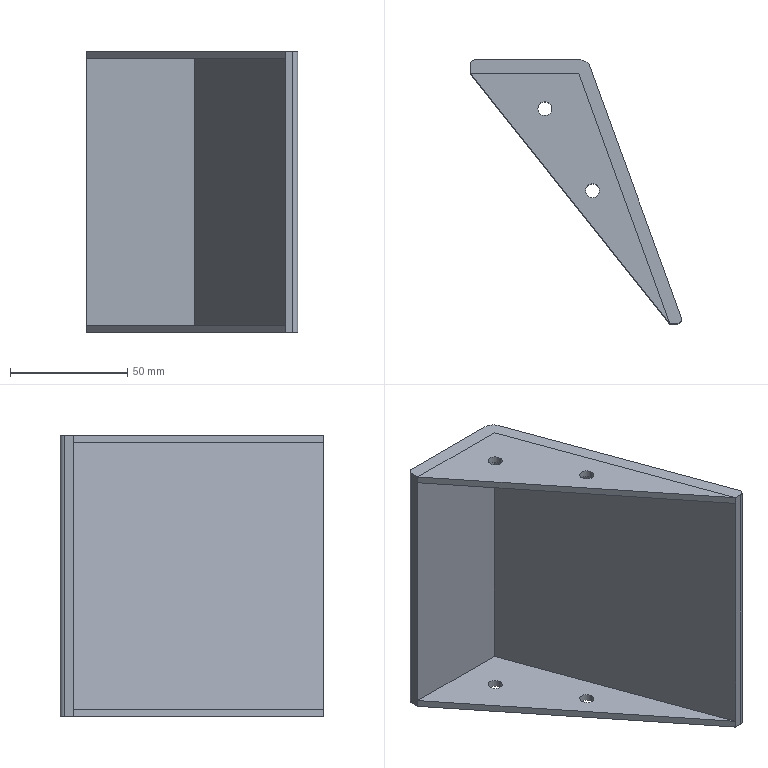Component | SolidWorks | Baffle-1 | 3 solids | 29 faces | box 90.19 x 112.76 x 120 mm | volume 125488 mm3 | plane 18 | cylinder 11 | commonest cylinder face diameters 6 x8 4 x2 10 x1
build123d program:
from build123d import *

# Parameters (mm, degrees)
BOSS_EXTRUDE1_DEPTH     = 120
BOSS_EXTRUDE2_DEPTH     = 3
FILLET2_R               = 5
FILLET4_R               = 2
CUT_EXTRUDE1_DEPTH      = 170
CUT_EXTRUDE1_DEPTH_BACK = 171.013
SKETCH3_R               = 3
BOSS_EXTRUDE3_DEPTH     = 3
SKETCH5_R               = 3
CUT_EXTRUDE2_DEPTH      = 173.092


with BuildPart() as part:
    # Sketch1 → Boss-Extrude1 (new body)
    with BuildSketch(Plane(origin=(0, 0, 0), x_dir=(0, 0, -1), z_dir=(1, 0, 0))):
        Polygon((-50, 0), (0, 0), (41.042, -112.763), (35.155, -112.763), (-3.745, -5.888), (-50, -5.888), align=None)
    extrude(amount=BOSS_EXTRUDE1_DEPTH)

    # Fillet2
    fillet2_edges = [part.edges().sort_by_distance(p)[0] for p in [
        (60, 0, 0),
    ]]
    fillet(fillet2_edges, radius=FILLET2_R)

    # Fillet4
    fillet4_edges = [part.edges().sort_by_distance(p)[0] for p in [
        (60, 0, 50),
        (60, -112.763, -41.042),
    ]]
    fillet(fillet4_edges, radius=FILLET4_R)


with BuildPart() as body_2:
    # Sketch2 → Boss-Extrude2 (new body)
    with BuildSketch(Plane.ZY):
        Polygon((-35.155, -112.763), (50, -5.888), (3.745, -5.888), align=None)
    extrude(amount=-BOSS_EXTRUDE2_DEPTH)

    # Sketch3 → Cut-Extrude1 (cut, two sides: drawn at the far end of the back side and taken through both)
    with BuildSketch(Plane(origin=(3, 0, 0), x_dir=(0, 0, -1), z_dir=(1, 0, 0)).offset(-CUT_EXTRUDE1_DEPTH_BACK)):
        with Locations((-18.169, -20.883)):
            Circle(SKETCH3_R)
        with Locations((2.146, -55.888)):
            Circle(SKETCH3_R)
    extrude(amount=CUT_EXTRUDE1_DEPTH + CUT_EXTRUDE1_DEPTH_BACK, mode=Mode.SUBTRACT)


with BuildPart() as body_3:
    # Sketch4 → Boss-Extrude3 (new body)
    with BuildSketch(Plane(origin=(120, 0, 0), x_dir=(0, 0, -1), z_dir=(1, 0, 0))):
        Polygon((-50, -5.888), (-3.745, -5.888), (35.155, -112.763), align=None)
    extrude(amount=-BOSS_EXTRUDE3_DEPTH)

    # Sketch5 → Cut-Extrude2 (cut, through all)
    with BuildSketch(Plane.ZY):
        with Locations((18.169, -20.883)):
            Circle(SKETCH5_R)
        with Locations((-2.146, -55.888)):
            Circle(SKETCH5_R)
    extrude(amount=-CUT_EXTRUDE2_DEPTH, mode=Mode.SUBTRACT)


solid = Compound([part.part, body_2.part, body_3.part])

# Placed as in the assembly
solid = solid.moved(Location((234.241, -164.715, 1470.724), (0, -90, 0)))
STEP:
#1=CARTESIAN_POINT('',(7.254,-6.564,62.627));
#2=VERTEX_POINT('',#1);
#3=CARTESIAN_POINT('',(7.254,-6.717,62.627));
#4=VERTEX_POINT('',#3);
#5=CARTESIAN_POINT('',(7.254,-6.485,62.627));
#6=DIRECTION('',(0.,-1.,0.));
#7=VECTOR('',#6,39.37);
#8=LINE('',#5,#7);
#9=EDGE_CURVE('',#2,#4,#8,.T.);
#10=ORIENTED_EDGE('',*,*,#9,.F.);
#11=CARTESIAN_POINT('',(7.254,-6.564,57.903));
#12=VERTEX_POINT('',#11);
#13=CARTESIAN_POINT('',(7.254,-6.564,62.627));
#14=DIRECTION('',(0.,0.,-1.));
#15=VECTOR('',#14,39.37);
#16=LINE('',#13,#15);
#17=EDGE_CURVE('',#2,#12,#16,.T.);
#18=ORIENTED_EDGE('',*,*,#17,.T.);
#19=CARTESIAN_POINT('',(7.254,-6.717,57.903));
#20=VERTEX_POINT('',#19);
#21=CARTESIAN_POINT('',(7.254,-6.485,57.903));
#22=DIRECTION('',(0.,-1.,0.));
#23=VECTOR('',#22,39.37);
#24=LINE('',#21,#23);
#25=EDGE_CURVE('',#12,#20,#24,.T.);
#26=ORIENTED_EDGE('',*,*,#25,.T.);
#27=CARTESIAN_POINT('',(7.254,-6.717,62.627));
#28=DIRECTION('',(0.,0.,-1.));
#29=VECTOR('',#28,39.37);
#30=LINE('',#27,#29);
#31=EDGE_CURVE('',#4,#20,#30,.T.);
#32=ORIENTED_EDGE('',*,*,#31,.F.);
#33=EDGE_LOOP('',(#10,#18,#26,#32));
#34=FACE_OUTER_BOUND('',#33,.T.);
#35=CARTESIAN_POINT('',(7.254,-6.485,62.627));
#36=DIRECTION('',(1.,0.,0.));
#37=DIRECTION('',(0.,0.,-1.));
#38=AXIS2_PLACEMENT_3D('',#35,#36,#37);
#39=PLANE('',#38);
#40=ADVANCED_FACE('',(#34),#39,.F.);
#41=CARTESIAN_POINT('',(9.075,-6.717,57.903));
#42=VERTEX_POINT('',#41);
#43=CARTESIAN_POINT('',(7.254,-6.717,57.903));
#44=DIRECTION('',(1.,0.,0.));
#45=VECTOR('',#44,39.37);
#46=LINE('',#43,#45);
#47=EDGE_CURVE('',#20,#42,#46,.T.);
#48=ORIENTED_EDGE('',*,*,#47,.T.);
#49=CARTESIAN_POINT('',(9.075,-6.717,62.627));
#50=VERTEX_POINT('',#49);
#51=CARTESIAN_POINT('',(9.075,-6.717,62.627));
#52=DIRECTION('',(0.,0.,-1.));
#53=VECTOR('',#52,39.37);
#54=LINE('',#51,#53);
#55=EDGE_CURVE('',#50,#42,#54,.T.);
#56=ORIENTED_EDGE('',*,*,#55,.F.);
#57=CARTESIAN_POINT('',(7.254,-6.717,62.627));
#58=DIRECTION('',(1.,0.,0.));
#59=VECTOR('',#58,39.37);
#60=LINE('',#57,#59);
#61=EDGE_CURVE('',#4,#50,#60,.T.);
#62=ORIENTED_EDGE('',*,*,#61,.F.);
#63=ORIENTED_EDGE('',*,*,#31,.T.);
#64=EDGE_LOOP('',(#48,#56,#62,#63));
#65=FACE_OUTER_BOUND('',#64,.T.);
#66=CARTESIAN_POINT('',(7.254,-6.717,62.627));
#67=DIRECTION('',(0.,1.,0.));
#68=DIRECTION('',(-1.,0.,0.));
#69=AXIS2_PLACEMENT_3D('',#66,#67,#68);
#70=PLANE('',#69);
#71=ADVANCED_FACE('',(#65),#70,.F.);
#72=CARTESIAN_POINT('',(10.606,-10.924,57.903));
#73=VERTEX_POINT('',#72);
#74=CARTESIAN_POINT('',(9.075,-6.717,57.903));
#75=DIRECTION('',(0.342,-0.9397,0.));
#76=VECTOR('',#75,39.37);
#77=LINE('',#74,#76);
#78=EDGE_CURVE('',#42,#73,#77,.T.);
#79=ORIENTED_EDGE('',*,*,#78,.T.);
#80=CARTESIAN_POINT('',(10.606,-10.924,62.627));
#81=VERTEX_POINT('',#80);
#82=CARTESIAN_POINT('',(10.606,-10.924,62.627));
#83=DIRECTION('',(0.,0.,-1.));
#84=VECTOR('',#83,39.37);
#85=LINE('',#82,#84);
#86=EDGE_CURVE('',#81,#73,#85,.T.);
#87=ORIENTED_EDGE('',*,*,#86,.F.);
#88=CARTESIAN_POINT('',(9.075,-6.717,62.627));
#89=DIRECTION('',(0.342,-0.9397,0.));
#90=VECTOR('',#89,39.37);
#91=LINE('',#88,#90);
#92=EDGE_CURVE('',#50,#81,#91,.T.);
#93=ORIENTED_EDGE('',*,*,#92,.F.);
#94=ORIENTED_EDGE('',*,*,#55,.T.);
#95=EDGE_LOOP('',(#79,#87,#93,#94));
#96=FACE_OUTER_BOUND('',#95,.T.);
#97=CARTESIAN_POINT('',(9.075,-6.717,62.627));
#98=DIRECTION('',(0.9397,0.342,0.));
#99=DIRECTION('',(-0.342,0.9397,0.));
#100=AXIS2_PLACEMENT_3D('',#97,#98,#99);
#101=PLANE('',#100);
#102=ADVANCED_FACE('',(#96),#101,.F.);
#103=CARTESIAN_POINT('',(10.725,-10.924,57.903));
#104=VERTEX_POINT('',#103);
#105=CARTESIAN_POINT('',(10.606,-10.924,57.903));
#106=DIRECTION('',(1.,0.,0.));
#107=VECTOR('',#106,39.37);
#108=LINE('',#105,#107);
#109=EDGE_CURVE('',#73,#104,#108,.T.);
#110=ORIENTED_EDGE('',*,*,#109,.T.);
#111=CARTESIAN_POINT('',(10.725,-10.924,62.627));
#112=VERTEX_POINT('',#111);
#113=CARTESIAN_POINT('',(10.725,-10.924,62.627));
#114=DIRECTION('',(0.,0.,1.));
#115=VECTOR('',#114,39.37);
#116=LINE('',#113,#115);
#117=EDGE_CURVE('',#104,#112,#116,.T.);
#118=ORIENTED_EDGE('',*,*,#117,.T.);
#119=CARTESIAN_POINT('',(10.606,-10.924,62.627));
#120=DIRECTION('',(1.,0.,0.));
#121=VECTOR('',#120,39.37);
#122=LINE('',#119,#121);
#123=EDGE_CURVE('',#81,#112,#122,.T.);
#124=ORIENTED_EDGE('',*,*,#123,.F.);
#125=ORIENTED_EDGE('',*,*,#86,.T.);
#126=EDGE_LOOP('',(#110,#118,#124,#125));
#127=FACE_OUTER_BOUND('',#126,.T.);
#128=CARTESIAN_POINT('',(10.606,-10.924,62.627));
#129=DIRECTION('',(0.,1.,0.));
#130=DIRECTION('',(-1.,0.,0.));
#131=AXIS2_PLACEMENT_3D('',#128,#129,#130);
#132=PLANE('',#131);
#133=ADVANCED_FACE('',(#127),#132,.F.);
#134=CARTESIAN_POINT('',(10.799,-10.819,62.627));
#135=VERTEX_POINT('',#134);
#136=CARTESIAN_POINT('',(9.269,-6.614,62.627));
#137=VERTEX_POINT('',#136);
#138=CARTESIAN_POINT('',(9.222,-6.485,62.627));
#139=DIRECTION('',(-0.342,0.9397,0.));
#140=VECTOR('',#139,39.37);
#141=LINE('',#138,#140);
#142=EDGE_CURVE('',#135,#137,#141,.T.);
#143=ORIENTED_EDGE('',*,*,#142,.F.);
#144=CARTESIAN_POINT('',(10.799,-10.819,57.903));
#145=VERTEX_POINT('',#144);
#146=CARTESIAN_POINT('',(10.799,-10.819,62.627));
#147=DIRECTION('',(0.,0.,-1.));
#148=VECTOR('',#147,39.37);
#149=LINE('',#146,#148);
#150=EDGE_CURVE('',#135,#145,#149,.T.);
#151=ORIENTED_EDGE('',*,*,#150,.T.);
#152=CARTESIAN_POINT('',(9.269,-6.614,57.903));
#153=VERTEX_POINT('',#152);
#154=CARTESIAN_POINT('',(9.222,-6.485,57.903));
#155=DIRECTION('',(-0.342,0.9397,0.));
#156=VECTOR('',#155,39.37);
#157=LINE('',#154,#156);
#158=EDGE_CURVE('',#145,#153,#157,.T.);
#159=ORIENTED_EDGE('',*,*,#158,.T.);
#160=CARTESIAN_POINT('',(9.269,-6.614,62.627));
#161=DIRECTION('',(0.,0.,1.));
#162=VECTOR('',#161,39.37);
#163=LINE('',#160,#162);
#164=EDGE_CURVE('',#153,#137,#163,.T.);
#165=ORIENTED_EDGE('',*,*,#164,.T.);
#166=EDGE_LOOP('',(#143,#151,#159,#165));
#167=FACE_OUTER_BOUND('',#166,.T.);
#168=CARTESIAN_POINT('',(9.222,-6.485,62.627));
#169=DIRECTION('',(-0.9397,-0.342,0.));
#170=DIRECTION('',(0.342,-0.9397,0.));
#171=AXIS2_PLACEMENT_3D('',#168,#169,#170);
#172=PLANE('',#171);
#173=ADVANCED_FACE('',(#167),#172,.F.);
#174=CARTESIAN_POINT('',(9.084,-6.485,57.903));
#175=VERTEX_POINT('',#174);
#176=CARTESIAN_POINT('',(7.332,-6.485,57.903));
#177=VERTEX_POINT('',#176);
#178=CARTESIAN_POINT('',(7.254,-6.485,57.903));
#179=DIRECTION('',(-1.,0.,0.));
#180=VECTOR('',#179,39.37);
#181=LINE('',#178,#180);
#182=EDGE_CURVE('',#175,#177,#181,.T.);
#183=ORIENTED_EDGE('',*,*,#182,.T.);
#184=CARTESIAN_POINT('',(7.332,-6.485,62.627));
#185=VERTEX_POINT('',#184);
#186=CARTESIAN_POINT('',(7.332,-6.485,62.627));
#187=DIRECTION('',(0.,0.,1.));
#188=VECTOR('',#187,39.37);
#189=LINE('',#186,#188);
#190=EDGE_CURVE('',#177,#185,#189,.T.);
#191=ORIENTED_EDGE('',*,*,#190,.T.);
#192=CARTESIAN_POINT('',(9.084,-6.485,62.627));
#193=VERTEX_POINT('',#192);
#194=CARTESIAN_POINT('',(7.254,-6.485,62.627));
#195=DIRECTION('',(-1.,0.,0.));
#196=VECTOR('',#195,39.37);
#197=LINE('',#194,#196);
#198=EDGE_CURVE('',#193,#185,#197,.T.);
#199=ORIENTED_EDGE('',*,*,#198,.F.);
#200=CARTESIAN_POINT('',(9.084,-6.485,62.627));
#201=DIRECTION('',(0.,0.,-1.));
#202=VECTOR('',#201,39.37);
#203=LINE('',#200,#202);
#204=EDGE_CURVE('',#193,#175,#203,.T.);
#205=ORIENTED_EDGE('',*,*,#204,.T.);
#206=EDGE_LOOP('',(#183,#191,#199,#205));
#207=FACE_OUTER_BOUND('',#206,.T.);
#208=CARTESIAN_POINT('',(7.254,-6.485,62.627));
#209=DIRECTION('',(0.,-1.,0.));
#210=DIRECTION('',(1.,0.,0.));
#211=AXIS2_PLACEMENT_3D('',#208,#209,#210);
#212=PLANE('',#211);
#213=ADVANCED_FACE('',(#207),#212,.F.);
#214=ORIENTED_EDGE('',*,*,#123,.T.);
#215=CARTESIAN_POINT('',(10.725,-10.846,62.627));
#216=DIRECTION('',(0.,0.,1.));
#217=DIRECTION('',(1.,0.,0.));
#218=AXIS2_PLACEMENT_3D('',#215,#216,#217);
#219=CIRCLE('',#218,0.07874);
#220=EDGE_CURVE('',#112,#135,#219,.T.);
#221=ORIENTED_EDGE('',*,*,#220,.T.);
#222=ORIENTED_EDGE('',*,*,#142,.T.);
#223=CARTESIAN_POINT('',(9.084,-6.682,62.627));
#224=DIRECTION('',(0.,0.,1.));
#225=DIRECTION('',(1.,0.,0.));
#226=AXIS2_PLACEMENT_3D('',#223,#224,#225);
#227=CIRCLE('',#226,0.1969);
#228=EDGE_CURVE('',#137,#193,#227,.T.);
#229=ORIENTED_EDGE('',*,*,#228,.T.);
#230=ORIENTED_EDGE('',*,*,#198,.T.);
#231=CARTESIAN_POINT('',(7.332,-6.564,62.627));
#232=DIRECTION('',(0.,0.,1.));
#233=DIRECTION('',(1.,0.,0.));
#234=AXIS2_PLACEMENT_3D('',#231,#232,#233);
#235=CIRCLE('',#234,0.07874);
#236=EDGE_CURVE('',#185,#2,#235,.T.);
#237=ORIENTED_EDGE('',*,*,#236,.T.);
#238=ORIENTED_EDGE('',*,*,#9,.T.);
#239=ORIENTED_EDGE('',*,*,#61,.T.);
#240=ORIENTED_EDGE('',*,*,#92,.T.);
#241=EDGE_LOOP('',(#214,#221,#222,#229,#230,#237,#238,#239,#240));
#242=FACE_OUTER_BOUND('',#241,.T.);
#243=CARTESIAN_POINT('',(9.222,-6.485,62.627));
#244=DIRECTION('',(0.,0.,1.));
#245=DIRECTION('',(1.,0.,0.));
#246=AXIS2_PLACEMENT_3D('',#243,#244,#245);
#247=PLANE('',#246);
#248=ADVANCED_FACE('',(#242),#247,.T.);
#249=ORIENTED_EDGE('',*,*,#158,.F.);
#250=CARTESIAN_POINT('',(10.725,-10.846,57.903));
#251=DIRECTION('',(0.,0.,-1.));
#252=DIRECTION('',(1.,0.,0.));
#253=AXIS2_PLACEMENT_3D('',#250,#251,#252);
#254=CIRCLE('',#253,0.07874);
#255=EDGE_CURVE('',#145,#104,#254,.T.);
#256=ORIENTED_EDGE('',*,*,#255,.T.);
#257=ORIENTED_EDGE('',*,*,#109,.F.);
#258=ORIENTED_EDGE('',*,*,#78,.F.);
#259=ORIENTED_EDGE('',*,*,#47,.F.);
#260=ORIENTED_EDGE('',*,*,#25,.F.);
#261=CARTESIAN_POINT('',(7.332,-6.564,57.903));
#262=DIRECTION('',(0.,0.,-1.));
#263=DIRECTION('',(1.,0.,0.));
#264=AXIS2_PLACEMENT_3D('',#261,#262,#263);
#265=CIRCLE('',#264,0.07874);
#266=EDGE_CURVE('',#12,#177,#265,.T.);
#267=ORIENTED_EDGE('',*,*,#266,.T.);
#268=ORIENTED_EDGE('',*,*,#182,.F.);
#269=CARTESIAN_POINT('',(9.084,-6.682,57.903));
#270=DIRECTION('',(0.,0.,-1.));
#271=DIRECTION('',(1.,0.,0.));
#272=AXIS2_PLACEMENT_3D('',#269,#270,#271);
#273=CIRCLE('',#272,0.1969);
#274=EDGE_CURVE('',#175,#153,#273,.T.);
#275=ORIENTED_EDGE('',*,*,#274,.T.);
#276=EDGE_LOOP('',(#249,#256,#257,#258,#259,#260,#267,#268,#275));
#277=FACE_OUTER_BOUND('',#276,.T.);
#278=CARTESIAN_POINT('',(9.222,-6.485,57.903));
#279=DIRECTION('',(0.,0.,1.));
#280=DIRECTION('',(1.,0.,0.));
#281=AXIS2_PLACEMENT_3D('',#278,#279,#280);
#282=PLANE('',#281);
#283=ADVANCED_FACE('',(#277),#282,.F.);
#284=ORIENTED_EDGE('',*,*,#228,.F.);
#285=ORIENTED_EDGE('',*,*,#164,.F.);
#286=ORIENTED_EDGE('',*,*,#274,.F.);
#287=ORIENTED_EDGE('',*,*,#204,.F.);
#288=EDGE_LOOP('',(#284,#285,#286,#287));
#289=FACE_OUTER_BOUND('',#288,.T.);
#290=CARTESIAN_POINT('',(9.084,-6.682,62.627));
#291=DIRECTION('',(0.,0.,-1.));
#292=DIRECTION('',(-1.,0.,0.));
#293=AXIS2_PLACEMENT_3D('',#290,#291,#292);
#294=CYLINDRICAL_SURFACE('',#293,0.1969);
#295=ADVANCED_FACE('',(#289),#294,.T.);
#296=ORIENTED_EDGE('',*,*,#220,.F.);
#297=ORIENTED_EDGE('',*,*,#117,.F.);
#298=ORIENTED_EDGE('',*,*,#255,.F.);
#299=ORIENTED_EDGE('',*,*,#150,.F.);
#300=EDGE_LOOP('',(#296,#297,#298,#299));
#301=FACE_OUTER_BOUND('',#300,.T.);
#302=CARTESIAN_POINT('',(10.725,-10.846,62.627));
#303=DIRECTION('',(0.,0.,-1.));
#304=DIRECTION('',(-1.,0.,0.));
#305=AXIS2_PLACEMENT_3D('',#302,#303,#304);
#306=CYLINDRICAL_SURFACE('',#305,0.07874);
#307=ADVANCED_FACE('',(#301),#306,.T.);
#308=ORIENTED_EDGE('',*,*,#236,.F.);
#309=ORIENTED_EDGE('',*,*,#190,.F.);
#310=ORIENTED_EDGE('',*,*,#266,.F.);
#311=ORIENTED_EDGE('',*,*,#17,.F.);
#312=EDGE_LOOP('',(#308,#309,#310,#311));
#313=FACE_OUTER_BOUND('',#312,.T.);
#314=CARTESIAN_POINT('',(7.332,-6.564,62.627));
#315=DIRECTION('',(0.,0.,-1.));
#316=DIRECTION('',(-1.,0.,0.));
#317=AXIS2_PLACEMENT_3D('',#314,#315,#316);
#318=CYLINDRICAL_SURFACE('',#317,0.07874);
#319=ADVANCED_FACE('',(#313),#318,.T.);
#320=CLOSED_SHELL('',(#40,#71,#102,#133,#173,#213,#248,#283,#295,#307,#319));
#321=MANIFOLD_SOLID_BREP('',#320);
#322=CARTESIAN_POINT('',(9.425,-8.685,62.627));
#323=VERTEX_POINT('',#322);
#324=CARTESIAN_POINT('',(9.188,-8.685,62.627));
#325=VERTEX_POINT('',#324);
#326=CARTESIAN_POINT('',(9.307,-8.685,62.627));
#327=DIRECTION('',(0.,0.,-1.));
#328=DIRECTION('',(-1.,0.,0.));
#329=AXIS2_PLACEMENT_3D('',#326,#327,#328);
#330=CIRCLE('',#329,0.1181);
#331=EDGE_CURVE('',#323,#325,#330,.T.);
#332=ORIENTED_EDGE('',*,*,#331,.F.);
#333=CARTESIAN_POINT('',(9.425,-8.685,62.509));
#334=VERTEX_POINT('',#333);
#335=CARTESIAN_POINT('',(9.425,-8.685,62.627));
#336=DIRECTION('',(0.,0.,-1.));
#337=VECTOR('',#336,39.37);
#338=LINE('',#335,#337);
#339=EDGE_CURVE('',#323,#334,#338,.T.);
#340=ORIENTED_EDGE('',*,*,#339,.T.);
#341=CARTESIAN_POINT('',(9.188,-8.685,62.509));
#342=VERTEX_POINT('',#341);
#343=CARTESIAN_POINT('',(9.307,-8.685,62.509));
#344=DIRECTION('',(0.,0.,-1.));
#345=DIRECTION('',(-1.,0.,0.));
#346=AXIS2_PLACEMENT_3D('',#343,#344,#345);
#347=CIRCLE('',#346,0.1181);
#348=EDGE_CURVE('',#334,#342,#347,.T.);
#349=ORIENTED_EDGE('',*,*,#348,.T.);
#350=CARTESIAN_POINT('',(9.188,-8.685,62.627));
#351=DIRECTION('',(0.,0.,-1.));
#352=VECTOR('',#351,39.37);
#353=LINE('',#350,#352);
#354=EDGE_CURVE('',#325,#342,#353,.T.);
#355=ORIENTED_EDGE('',*,*,#354,.F.);
#356=EDGE_LOOP('',(#332,#340,#349,#355));
#357=FACE_OUTER_BOUND('',#356,.T.);
#358=CARTESIAN_POINT('',(9.307,-8.685,62.627));
#359=DIRECTION('',(0.,0.,-1.));
#360=DIRECTION('',(-1.,0.,0.));
#361=AXIS2_PLACEMENT_3D('',#358,#359,#360);
#362=CYLINDRICAL_SURFACE('',#361,0.1181);
#363=ADVANCED_FACE('',(#357),#362,.F.);
#364=CARTESIAN_POINT('',(8.625,-7.307,62.627));
#365=VERTEX_POINT('',#364);
#366=CARTESIAN_POINT('',(8.389,-7.307,62.627));
#367=VERTEX_POINT('',#366);
#368=CARTESIAN_POINT('',(8.507,-7.307,62.627));
#369=DIRECTION('',(0.,0.,-1.));
#370=DIRECTION('',(-1.,0.,0.));
#371=AXIS2_PLACEMENT_3D('',#368,#369,#370);
#372=CIRCLE('',#371,0.1181);
#373=EDGE_CURVE('',#365,#367,#372,.T.);
#374=ORIENTED_EDGE('',*,*,#373,.F.);
#375=CARTESIAN_POINT('',(8.625,-7.307,62.509));
#376=VERTEX_POINT('',#375);
#377=CARTESIAN_POINT('',(8.625,-7.307,62.627));
#378=DIRECTION('',(0.,0.,-1.));
#379=VECTOR('',#378,39.37);
#380=LINE('',#377,#379);
#381=EDGE_CURVE('',#365,#376,#380,.T.);
#382=ORIENTED_EDGE('',*,*,#381,.T.);
#383=CARTESIAN_POINT('',(8.389,-7.307,62.509));
#384=VERTEX_POINT('',#383);
#385=CARTESIAN_POINT('',(8.507,-7.307,62.509));
#386=DIRECTION('',(0.,0.,-1.));
#387=DIRECTION('',(-1.,0.,0.));
#388=AXIS2_PLACEMENT_3D('',#385,#386,#387);
#389=CIRCLE('',#388,0.1181);
#390=EDGE_CURVE('',#376,#384,#389,.T.);
#391=ORIENTED_EDGE('',*,*,#390,.T.);
#392=CARTESIAN_POINT('',(8.389,-7.307,62.627));
#393=DIRECTION('',(0.,0.,-1.));
#394=VECTOR('',#393,39.37);
#395=LINE('',#392,#394);
#396=EDGE_CURVE('',#367,#384,#395,.T.);
#397=ORIENTED_EDGE('',*,*,#396,.F.);
#398=EDGE_LOOP('',(#374,#382,#391,#397));
#399=FACE_OUTER_BOUND('',#398,.T.);
#400=CARTESIAN_POINT('',(8.507,-7.307,62.627));
#401=DIRECTION('',(0.,0.,-1.));
#402=DIRECTION('',(-1.,0.,0.));
#403=AXIS2_PLACEMENT_3D('',#400,#401,#402);
#404=CYLINDRICAL_SURFACE('',#403,0.1181);
#405=ADVANCED_FACE('',(#399),#404,.F.);
#406=CARTESIAN_POINT('',(7.254,-6.717,62.627));
#407=VERTEX_POINT('',#406);
#408=CARTESIAN_POINT('',(10.606,-10.924,62.627));
#409=VERTEX_POINT('',#408);
#410=CARTESIAN_POINT('',(10.606,-10.924,62.627));
#411=DIRECTION('',(0.6232,-0.7821,0.));
#412=VECTOR('',#411,39.37);
#413=LINE('',#410,#412);
#414=EDGE_CURVE('',#407,#409,#413,.T.);
#415=ORIENTED_EDGE('',*,*,#414,.F.);
#416=CARTESIAN_POINT('',(7.254,-6.717,62.509));
#417=VERTEX_POINT('',#416);
#418=CARTESIAN_POINT('',(7.254,-6.717,62.509));
#419=DIRECTION('',(0.,0.,1.));
#420=VECTOR('',#419,39.37);
#421=LINE('',#418,#420);
#422=EDGE_CURVE('',#417,#407,#421,.T.);
#423=ORIENTED_EDGE('',*,*,#422,.F.);
#424=CARTESIAN_POINT('',(10.606,-10.924,62.509));
#425=VERTEX_POINT('',#424);
#426=CARTESIAN_POINT('',(10.606,-10.924,62.509));
#427=DIRECTION('',(0.6232,-0.7821,0.));
#428=VECTOR('',#427,39.37);
#429=LINE('',#426,#428);
#430=EDGE_CURVE('',#417,#425,#429,.T.);
#431=ORIENTED_EDGE('',*,*,#430,.T.);
#432=CARTESIAN_POINT('',(10.606,-10.924,62.509));
#433=DIRECTION('',(0.,0.,1.));
#434=VECTOR('',#433,39.37);
#435=LINE('',#432,#434);
#436=EDGE_CURVE('',#425,#409,#435,.T.);
#437=ORIENTED_EDGE('',*,*,#436,.T.);
#438=EDGE_LOOP('',(#415,#423,#431,#437));
#439=FACE_OUTER_BOUND('',#438,.T.);
#440=CARTESIAN_POINT('',(10.606,-10.924,62.509));
#441=DIRECTION('',(-0.7821,-0.6232,0.));
#442=DIRECTION('',(0.6232,-0.7821,0.));
#443=AXIS2_PLACEMENT_3D('',#440,#441,#442);
#444=PLANE('',#443);
#445=ADVANCED_FACE('',(#439),#444,.T.);
#446=CARTESIAN_POINT('',(9.075,-6.717,62.627));
#447=VERTEX_POINT('',#446);
#448=CARTESIAN_POINT('',(7.254,-6.717,62.627));
#449=DIRECTION('',(-1.,0.,0.));
#450=VECTOR('',#449,39.37);
#451=LINE('',#448,#450);
#452=EDGE_CURVE('',#447,#407,#451,.T.);
#453=ORIENTED_EDGE('',*,*,#452,.F.);
#454=CARTESIAN_POINT('',(9.075,-6.717,62.509));
#455=VERTEX_POINT('',#454);
#456=CARTESIAN_POINT('',(9.075,-6.717,62.509));
#457=DIRECTION('',(0.,0.,1.));
#458=VECTOR('',#457,39.37);
#459=LINE('',#456,#458);
#460=EDGE_CURVE('',#455,#447,#459,.T.);
#461=ORIENTED_EDGE('',*,*,#460,.F.);
#462=CARTESIAN_POINT('',(7.254,-6.717,62.509));
#463=DIRECTION('',(-1.,0.,0.));
#464=VECTOR('',#463,39.37);
#465=LINE('',#462,#464);
#466=EDGE_CURVE('',#455,#417,#465,.T.);
#467=ORIENTED_EDGE('',*,*,#466,.T.);
#468=ORIENTED_EDGE('',*,*,#422,.T.);
#469=EDGE_LOOP('',(#453,#461,#467,#468));
#470=FACE_OUTER_BOUND('',#469,.T.);
#471=CARTESIAN_POINT('',(7.254,-6.717,62.509));
#472=DIRECTION('',(0.,1.,0.));
#473=DIRECTION('',(-1.,0.,0.));
#474=AXIS2_PLACEMENT_3D('',#471,#472,#473);
#475=PLANE('',#474);
#476=ADVANCED_FACE('',(#470),#475,.T.);
#477=CARTESIAN_POINT('',(9.075,-6.717,62.627));
#478=DIRECTION('',(-0.342,0.9397,0.));
#479=VECTOR('',#478,39.37);
#480=LINE('',#477,#479);
#481=EDGE_CURVE('',#409,#447,#480,.T.);
#482=ORIENTED_EDGE('',*,*,#481,.F.);
#483=ORIENTED_EDGE('',*,*,#436,.F.);
#484=CARTESIAN_POINT('',(9.075,-6.717,62.509));
#485=DIRECTION('',(-0.342,0.9397,0.));
#486=VECTOR('',#485,39.37);
#487=LINE('',#484,#486);
#488=EDGE_CURVE('',#425,#455,#487,.T.);
#489=ORIENTED_EDGE('',*,*,#488,.T.);
#490=ORIENTED_EDGE('',*,*,#460,.T.);
#491=EDGE_LOOP('',(#482,#483,#489,#490));
#492=FACE_OUTER_BOUND('',#491,.T.);
#493=CARTESIAN_POINT('',(9.075,-6.717,62.509));
#494=DIRECTION('',(0.9397,0.342,0.));
#495=DIRECTION('',(-0.342,0.9397,0.));
#496=AXIS2_PLACEMENT_3D('',#493,#494,#495);
#497=PLANE('',#496);
#498=ADVANCED_FACE('',(#492),#497,.T.);
#499=CARTESIAN_POINT('',(9.307,-8.685,62.509));
#500=DIRECTION('',(0.,0.,-1.));
#501=DIRECTION('',(-1.,0.,0.));
#502=AXIS2_PLACEMENT_3D('',#499,#500,#501);
#503=CIRCLE('',#502,0.1181);
#504=EDGE_CURVE('',#342,#334,#503,.T.);
#505=ORIENTED_EDGE('',*,*,#504,.F.);
#506=ORIENTED_EDGE('',*,*,#348,.F.);
#507=EDGE_LOOP('',(#505,#506));
#508=FACE_BOUND('',#507,.T.);
#509=CARTESIAN_POINT('',(8.507,-7.307,62.509));
#510=DIRECTION('',(0.,0.,-1.));
#511=DIRECTION('',(-1.,0.,0.));
#512=AXIS2_PLACEMENT_3D('',#509,#510,#511);
#513=CIRCLE('',#512,0.1181);
#514=EDGE_CURVE('',#384,#376,#513,.T.);
#515=ORIENTED_EDGE('',*,*,#514,.F.);
#516=ORIENTED_EDGE('',*,*,#390,.F.);
#517=EDGE_LOOP('',(#515,#516));
#518=FACE_BOUND('',#517,.T.);
#519=ORIENTED_EDGE('',*,*,#430,.F.);
#520=ORIENTED_EDGE('',*,*,#466,.F.);
#521=ORIENTED_EDGE('',*,*,#488,.F.);
#522=EDGE_LOOP('',(#519,#520,#521));
#523=FACE_OUTER_BOUND('',#522,.T.);
#524=CARTESIAN_POINT('',(9.222,-6.485,62.509));
#525=DIRECTION('',(0.,0.,-1.));
#526=DIRECTION('',(-1.,0.,0.));
#527=AXIS2_PLACEMENT_3D('',#524,#525,#526);
#528=PLANE('',#527);
#529=ADVANCED_FACE('',(#508,#518,#523),#528,.T.);
#530=CARTESIAN_POINT('',(9.307,-8.685,62.627));
#531=DIRECTION('',(0.,0.,-1.));
#532=DIRECTION('',(-1.,0.,0.));
#533=AXIS2_PLACEMENT_3D('',#530,#531,#532);
#534=CIRCLE('',#533,0.1181);
#535=EDGE_CURVE('',#325,#323,#534,.T.);
#536=ORIENTED_EDGE('',*,*,#535,.T.);
#537=ORIENTED_EDGE('',*,*,#331,.T.);
#538=EDGE_LOOP('',(#536,#537));
#539=FACE_BOUND('',#538,.T.);
#540=CARTESIAN_POINT('',(8.507,-7.307,62.627));
#541=DIRECTION('',(0.,0.,-1.));
#542=DIRECTION('',(-1.,0.,0.));
#543=AXIS2_PLACEMENT_3D('',#540,#541,#542);
#544=CIRCLE('',#543,0.1181);
#545=EDGE_CURVE('',#367,#365,#544,.T.);
#546=ORIENTED_EDGE('',*,*,#545,.T.);
#547=ORIENTED_EDGE('',*,*,#373,.T.);
#548=EDGE_LOOP('',(#546,#547));
#549=FACE_BOUND('',#548,.T.);
#550=ORIENTED_EDGE('',*,*,#414,.T.);
#551=ORIENTED_EDGE('',*,*,#481,.T.);
#552=ORIENTED_EDGE('',*,*,#452,.T.);
#553=EDGE_LOOP('',(#550,#551,#552));
#554=FACE_OUTER_BOUND('',#553,.T.);
#555=CARTESIAN_POINT('',(9.222,-6.485,62.627));
#556=DIRECTION('',(0.,0.,-1.));
#557=DIRECTION('',(-1.,0.,0.));
#558=AXIS2_PLACEMENT_3D('',#555,#556,#557);
#559=PLANE('',#558);
#560=ADVANCED_FACE('',(#539,#549,#554),#559,.F.);
#561=ORIENTED_EDGE('',*,*,#381,.F.);
#562=ORIENTED_EDGE('',*,*,#545,.F.);
#563=ORIENTED_EDGE('',*,*,#396,.T.);
#564=ORIENTED_EDGE('',*,*,#514,.T.);
#565=EDGE_LOOP('',(#561,#562,#563,#564));
#566=FACE_OUTER_BOUND('',#565,.T.);
#567=CARTESIAN_POINT('',(8.507,-7.307,62.627));
#568=DIRECTION('',(0.,0.,-1.));
#569=DIRECTION('',(-1.,0.,0.));
#570=AXIS2_PLACEMENT_3D('',#567,#568,#569);
#571=CYLINDRICAL_SURFACE('',#570,0.1181);
#572=ADVANCED_FACE('',(#566),#571,.F.);
#573=ORIENTED_EDGE('',*,*,#339,.F.);
#574=ORIENTED_EDGE('',*,*,#535,.F.);
#575=ORIENTED_EDGE('',*,*,#354,.T.);
#576=ORIENTED_EDGE('',*,*,#504,.T.);
#577=EDGE_LOOP('',(#573,#574,#575,#576));
#578=FACE_OUTER_BOUND('',#577,.T.);
#579=CARTESIAN_POINT('',(9.307,-8.685,62.627));
#580=DIRECTION('',(0.,0.,-1.));
#581=DIRECTION('',(-1.,0.,0.));
#582=AXIS2_PLACEMENT_3D('',#579,#580,#581);
#583=CYLINDRICAL_SURFACE('',#582,0.1181);
#584=ADVANCED_FACE('',(#578),#583,.F.);
#585=CLOSED_SHELL('',(#363,#405,#445,#476,#498,#529,#560,#572,#584));
#586=MANIFOLD_SOLID_BREP('',#585);
#587=CARTESIAN_POINT('',(9.425,-8.685,58.021));
#588=VERTEX_POINT('',#587);
#589=CARTESIAN_POINT('',(9.188,-8.685,58.021));
#590=VERTEX_POINT('',#589);
#591=CARTESIAN_POINT('',(9.307,-8.685,58.021));
#592=DIRECTION('',(0.,0.,-1.));
#593=DIRECTION('',(1.,0.,0.));
#594=AXIS2_PLACEMENT_3D('',#591,#592,#593);
#595=CIRCLE('',#594,0.1181);
#596=EDGE_CURVE('',#588,#590,#595,.T.);
#597=ORIENTED_EDGE('',*,*,#596,.F.);
#598=CARTESIAN_POINT('',(9.425,-8.685,57.903));
#599=VERTEX_POINT('',#598);
#600=CARTESIAN_POINT('',(9.425,-8.685,64.714));
#601=DIRECTION('',(0.,0.,-1.));
#602=VECTOR('',#601,39.37);
#603=LINE('',#600,#602);
#604=EDGE_CURVE('',#588,#599,#603,.T.);
#605=ORIENTED_EDGE('',*,*,#604,.T.);
#606=CARTESIAN_POINT('',(9.188,-8.685,57.903));
#607=VERTEX_POINT('',#606);
#608=CARTESIAN_POINT('',(9.307,-8.685,57.903));
#609=DIRECTION('',(0.,0.,1.));
#610=DIRECTION('',(1.,0.,0.));
#611=AXIS2_PLACEMENT_3D('',#608,#609,#610);
#612=CIRCLE('',#611,0.1181);
#613=EDGE_CURVE('',#607,#599,#612,.T.);
#614=ORIENTED_EDGE('',*,*,#613,.F.);
#615=CARTESIAN_POINT('',(9.188,-8.685,64.714));
#616=DIRECTION('',(0.,0.,-1.));
#617=VECTOR('',#616,39.37);
#618=LINE('',#615,#617);
#619=EDGE_CURVE('',#590,#607,#618,.T.);
#620=ORIENTED_EDGE('',*,*,#619,.F.);
#621=EDGE_LOOP('',(#597,#605,#614,#620));
#622=FACE_OUTER_BOUND('',#621,.T.);
#623=CARTESIAN_POINT('',(9.307,-8.685,64.714));
#624=DIRECTION('',(0.,0.,-1.));
#625=DIRECTION('',(-1.,0.,0.));
#626=AXIS2_PLACEMENT_3D('',#623,#624,#625);
#627=CYLINDRICAL_SURFACE('',#626,0.1181);
#628=ADVANCED_FACE('',(#622),#627,.F.);
#629=CARTESIAN_POINT('',(8.625,-7.307,58.021));
#630=VERTEX_POINT('',#629);
#631=CARTESIAN_POINT('',(8.389,-7.307,58.021));
#632=VERTEX_POINT('',#631);
#633=CARTESIAN_POINT('',(8.507,-7.307,58.021));
#634=DIRECTION('',(0.,0.,-1.));
#635=DIRECTION('',(1.,0.,0.));
#636=AXIS2_PLACEMENT_3D('',#633,#634,#635);
#637=CIRCLE('',#636,0.1181);
#638=EDGE_CURVE('',#630,#632,#637,.T.);
#639=ORIENTED_EDGE('',*,*,#638,.F.);
#640=CARTESIAN_POINT('',(8.625,-7.307,57.903));
#641=VERTEX_POINT('',#640);
#642=CARTESIAN_POINT('',(8.625,-7.307,64.714));
#643=DIRECTION('',(0.,0.,-1.));
#644=VECTOR('',#643,39.37);
#645=LINE('',#642,#644);
#646=EDGE_CURVE('',#630,#641,#645,.T.);
#647=ORIENTED_EDGE('',*,*,#646,.T.);
#648=CARTESIAN_POINT('',(8.389,-7.307,57.903));
#649=VERTEX_POINT('',#648);
#650=CARTESIAN_POINT('',(8.507,-7.307,57.903));
#651=DIRECTION('',(0.,0.,1.));
#652=DIRECTION('',(1.,0.,0.));
#653=AXIS2_PLACEMENT_3D('',#650,#651,#652);
#654=CIRCLE('',#653,0.1181);
#655=EDGE_CURVE('',#649,#641,#654,.T.);
#656=ORIENTED_EDGE('',*,*,#655,.F.);
#657=CARTESIAN_POINT('',(8.389,-7.307,64.714));
#658=DIRECTION('',(0.,0.,-1.));
#659=VECTOR('',#658,39.37);
#660=LINE('',#657,#659);
#661=EDGE_CURVE('',#632,#649,#660,.T.);
#662=ORIENTED_EDGE('',*,*,#661,.F.);
#663=EDGE_LOOP('',(#639,#647,#656,#662));
#664=FACE_OUTER_BOUND('',#663,.T.);
#665=CARTESIAN_POINT('',(8.507,-7.307,64.714));
#666=DIRECTION('',(0.,0.,-1.));
#667=DIRECTION('',(-1.,0.,0.));
#668=AXIS2_PLACEMENT_3D('',#665,#666,#667);
#669=CYLINDRICAL_SURFACE('',#668,0.1181);
#670=ADVANCED_FACE('',(#664),#669,.F.);
#671=CARTESIAN_POINT('',(8.507,-7.307,58.021));
#672=DIRECTION('',(0.,0.,-1.));
#673=DIRECTION('',(1.,0.,0.));
#674=AXIS2_PLACEMENT_3D('',#671,#672,#673);
#675=CIRCLE('',#674,0.1181);
#676=EDGE_CURVE('',#632,#630,#675,.T.);
#677=ORIENTED_EDGE('',*,*,#676,.T.);
#678=ORIENTED_EDGE('',*,*,#638,.T.);
#679=EDGE_LOOP('',(#677,#678));
#680=FACE_BOUND('',#679,.T.);
#681=CARTESIAN_POINT('',(9.075,-6.717,58.021));
#682=VERTEX_POINT('',#681);
#683=CARTESIAN_POINT('',(10.606,-10.924,58.021));
#684=VERTEX_POINT('',#683);
#685=CARTESIAN_POINT('',(9.075,-6.717,58.021));
#686=DIRECTION('',(0.342,-0.9397,0.));
#687=VECTOR('',#686,39.37);
#688=LINE('',#685,#687);
#689=EDGE_CURVE('',#682,#684,#688,.T.);
#690=ORIENTED_EDGE('',*,*,#689,.F.);
#691=CARTESIAN_POINT('',(7.254,-6.717,58.021));
#692=VERTEX_POINT('',#691);
#693=CARTESIAN_POINT('',(7.254,-6.717,58.021));
#694=DIRECTION('',(1.,0.,0.));
#695=VECTOR('',#694,39.37);
#696=LINE('',#693,#695);
#697=EDGE_CURVE('',#692,#682,#696,.T.);
#698=ORIENTED_EDGE('',*,*,#697,.F.);
#699=CARTESIAN_POINT('',(10.606,-10.924,58.021));
#700=DIRECTION('',(-0.6232,0.7821,0.));
#701=VECTOR('',#700,39.37);
#702=LINE('',#699,#701);
#703=EDGE_CURVE('',#684,#692,#702,.T.);
#704=ORIENTED_EDGE('',*,*,#703,.F.);
#705=EDGE_LOOP('',(#690,#698,#704));
#706=FACE_OUTER_BOUND('',#705,.T.);
#707=CARTESIAN_POINT('',(9.307,-8.685,58.021));
#708=DIRECTION('',(0.,0.,-1.));
#709=DIRECTION('',(1.,0.,0.));
#710=AXIS2_PLACEMENT_3D('',#707,#708,#709);
#711=CIRCLE('',#710,0.1181);
#712=EDGE_CURVE('',#590,#588,#711,.T.);
#713=ORIENTED_EDGE('',*,*,#712,.T.);
#714=ORIENTED_EDGE('',*,*,#596,.T.);
#715=EDGE_LOOP('',(#713,#714));
#716=FACE_BOUND('',#715,.T.);
#717=CARTESIAN_POINT('',(9.222,-6.485,58.021));
#718=DIRECTION('',(0.,0.,1.));
#719=DIRECTION('',(1.,0.,0.));
#720=AXIS2_PLACEMENT_3D('',#717,#718,#719);
#721=PLANE('',#720);
#722=ADVANCED_FACE('',(#680,#706,#716),#721,.T.);
#723=ORIENTED_EDGE('',*,*,#655,.T.);
#724=CARTESIAN_POINT('',(8.507,-7.307,57.903));
#725=DIRECTION('',(0.,0.,1.));
#726=DIRECTION('',(1.,0.,0.));
#727=AXIS2_PLACEMENT_3D('',#724,#725,#726);
#728=CIRCLE('',#727,0.1181);
#729=EDGE_CURVE('',#641,#649,#728,.T.);
#730=ORIENTED_EDGE('',*,*,#729,.T.);
#731=EDGE_LOOP('',(#723,#730));
#732=FACE_BOUND('',#731,.T.);
#733=CARTESIAN_POINT('',(9.075,-6.717,57.903));
#734=VERTEX_POINT('',#733);
#735=CARTESIAN_POINT('',(10.606,-10.924,57.903));
#736=VERTEX_POINT('',#735);
#737=CARTESIAN_POINT('',(9.075,-6.717,57.903));
#738=DIRECTION('',(0.342,-0.9397,0.));
#739=VECTOR('',#738,39.37);
#740=LINE('',#737,#739);
#741=EDGE_CURVE('',#734,#736,#740,.T.);
#742=ORIENTED_EDGE('',*,*,#741,.T.);
#743=CARTESIAN_POINT('',(7.254,-6.717,57.903));
#744=VERTEX_POINT('',#743);
#745=CARTESIAN_POINT('',(10.606,-10.924,57.903));
#746=DIRECTION('',(-0.6232,0.7821,0.));
#747=VECTOR('',#746,39.37);
#748=LINE('',#745,#747);
#749=EDGE_CURVE('',#736,#744,#748,.T.);
#750=ORIENTED_EDGE('',*,*,#749,.T.);
#751=CARTESIAN_POINT('',(7.254,-6.717,57.903));
#752=DIRECTION('',(1.,0.,0.));
#753=VECTOR('',#752,39.37);
#754=LINE('',#751,#753);
#755=EDGE_CURVE('',#744,#734,#754,.T.);
#756=ORIENTED_EDGE('',*,*,#755,.T.);
#757=EDGE_LOOP('',(#742,#750,#756));
#758=FACE_OUTER_BOUND('',#757,.T.);
#759=ORIENTED_EDGE('',*,*,#613,.T.);
#760=CARTESIAN_POINT('',(9.307,-8.685,57.903));
#761=DIRECTION('',(0.,0.,1.));
#762=DIRECTION('',(1.,0.,0.));
#763=AXIS2_PLACEMENT_3D('',#760,#761,#762);
#764=CIRCLE('',#763,0.1181);
#765=EDGE_CURVE('',#599,#607,#764,.T.);
#766=ORIENTED_EDGE('',*,*,#765,.T.);
#767=EDGE_LOOP('',(#759,#766));
#768=FACE_BOUND('',#767,.T.);
#769=CARTESIAN_POINT('',(9.222,-6.485,57.903));
#770=DIRECTION('',(0.,0.,1.));
#771=DIRECTION('',(1.,0.,0.));
#772=AXIS2_PLACEMENT_3D('',#769,#770,#771);
#773=PLANE('',#772);
#774=ADVANCED_FACE('',(#732,#758,#768),#773,.F.);
#775=ORIENTED_EDGE('',*,*,#741,.F.);
#776=CARTESIAN_POINT('',(9.075,-6.717,58.021));
#777=DIRECTION('',(0.,0.,-1.));
#778=VECTOR('',#777,39.37);
#779=LINE('',#776,#778);
#780=EDGE_CURVE('',#682,#734,#779,.T.);
#781=ORIENTED_EDGE('',*,*,#780,.F.);
#782=ORIENTED_EDGE('',*,*,#689,.T.);
#783=CARTESIAN_POINT('',(10.606,-10.924,58.021));
#784=DIRECTION('',(0.,0.,-1.));
#785=VECTOR('',#784,39.37);
#786=LINE('',#783,#785);
#787=EDGE_CURVE('',#684,#736,#786,.T.);
#788=ORIENTED_EDGE('',*,*,#787,.T.);
#789=EDGE_LOOP('',(#775,#781,#782,#788));
#790=FACE_OUTER_BOUND('',#789,.T.);
#791=CARTESIAN_POINT('',(9.075,-6.717,58.021));
#792=DIRECTION('',(0.9397,0.342,0.));
#793=DIRECTION('',(-0.342,0.9397,0.));
#794=AXIS2_PLACEMENT_3D('',#791,#792,#793);
#795=PLANE('',#794);
#796=ADVANCED_FACE('',(#790),#795,.T.);
#797=ORIENTED_EDGE('',*,*,#755,.F.);
#798=CARTESIAN_POINT('',(7.254,-6.717,58.021));
#799=DIRECTION('',(0.,0.,-1.));
#800=VECTOR('',#799,39.37);
#801=LINE('',#798,#800);
#802=EDGE_CURVE('',#692,#744,#801,.T.);
#803=ORIENTED_EDGE('',*,*,#802,.F.);
#804=ORIENTED_EDGE('',*,*,#697,.T.);
#805=ORIENTED_EDGE('',*,*,#780,.T.);
#806=EDGE_LOOP('',(#797,#803,#804,#805));
#807=FACE_OUTER_BOUND('',#806,.T.);
#808=CARTESIAN_POINT('',(7.254,-6.717,58.021));
#809=DIRECTION('',(0.,1.,0.));
#810=DIRECTION('',(-1.,0.,0.));
#811=AXIS2_PLACEMENT_3D('',#808,#809,#810);
#812=PLANE('',#811);
#813=ADVANCED_FACE('',(#807),#812,.T.);
#814=ORIENTED_EDGE('',*,*,#749,.F.);
#815=ORIENTED_EDGE('',*,*,#787,.F.);
#816=ORIENTED_EDGE('',*,*,#703,.T.);
#817=ORIENTED_EDGE('',*,*,#802,.T.);
#818=EDGE_LOOP('',(#814,#815,#816,#817));
#819=FACE_OUTER_BOUND('',#818,.T.);
#820=CARTESIAN_POINT('',(10.606,-10.924,58.021));
#821=DIRECTION('',(-0.7821,-0.6232,0.));
#822=DIRECTION('',(0.6232,-0.7821,0.));
#823=AXIS2_PLACEMENT_3D('',#820,#821,#822);
#824=PLANE('',#823);
#825=ADVANCED_FACE('',(#819),#824,.T.);
#826=ORIENTED_EDGE('',*,*,#646,.F.);
#827=ORIENTED_EDGE('',*,*,#676,.F.);
#828=ORIENTED_EDGE('',*,*,#661,.T.);
#829=ORIENTED_EDGE('',*,*,#729,.F.);
#830=EDGE_LOOP('',(#826,#827,#828,#829));
#831=FACE_OUTER_BOUND('',#830,.T.);
#832=CARTESIAN_POINT('',(8.507,-7.307,64.714));
#833=DIRECTION('',(0.,0.,-1.));
#834=DIRECTION('',(-1.,0.,0.));
#835=AXIS2_PLACEMENT_3D('',#832,#833,#834);
#836=CYLINDRICAL_SURFACE('',#835,0.1181);
#837=ADVANCED_FACE('',(#831),#836,.F.);
#838=ORIENTED_EDGE('',*,*,#604,.F.);
#839=ORIENTED_EDGE('',*,*,#712,.F.);
#840=ORIENTED_EDGE('',*,*,#619,.T.);
#841=ORIENTED_EDGE('',*,*,#765,.F.);
#842=EDGE_LOOP('',(#838,#839,#840,#841));
#843=FACE_OUTER_BOUND('',#842,.T.);
#844=CARTESIAN_POINT('',(9.307,-8.685,64.714));
#845=DIRECTION('',(0.,0.,-1.));
#846=DIRECTION('',(-1.,0.,0.));
#847=AXIS2_PLACEMENT_3D('',#844,#845,#846);
#848=CYLINDRICAL_SURFACE('',#847,0.1181);
#849=ADVANCED_FACE('',(#843),#848,.F.);
#850=CLOSED_SHELL('',(#628,#670,#722,#774,#796,#813,#825,#837,#849));
#851=MANIFOLD_SOLID_BREP('',#850);
#852=CARTESIAN_POINT('',(0.,0.,0.));
#853=DIRECTION('',(0.,0.,1.));
#854=DIRECTION('',(1.,0.,0.));
#855=AXIS2_PLACEMENT_3D('',#852,#853,#854);
#856=(LENGTH_UNIT()NAMED_UNIT(*)SI_UNIT($,.METRE.));
#857=LENGTH_MEASURE_WITH_UNIT(LENGTH_MEASURE(0.0254),#856);
#858=DIMENSIONAL_EXPONENTS(1.,0.,0.,0.,0.,0.,0.);
#859=(CONVERSION_BASED_UNIT('',#857)LENGTH_UNIT()NAMED_UNIT(#858));
#860=UNCERTAINTY_MEASURE_WITH_UNIT(LENGTH_MEASURE(0.00001),#859,'','');
#861=(NAMED_UNIT(*)PLANE_ANGLE_UNIT()SI_UNIT($,.RADIAN.));
#862=(NAMED_UNIT(*)SI_UNIT($,.STERADIAN.)SOLID_ANGLE_UNIT());
#863=(GEOMETRIC_REPRESENTATION_CONTEXT(3)GLOBAL_UNCERTAINTY_ASSIGNED_CONTEXT((#860))GLOBAL_UNIT_ASSIGNED_CONTEXT((#859,#861,#862))REPRESENTATION_CONTEXT('',''));
#864=ADVANCED_BREP_SHAPE_REPRESENTATION('',(#321,#586,#851,#855),#863);
#865=COLOUR_RGB('',0.7922,0.8196,0.9333);
#866=FILL_AREA_STYLE_COLOUR('',#865);
#867=FILL_AREA_STYLE('',(#866));
#868=SURFACE_STYLE_FILL_AREA(#867);
#869=SURFACE_SIDE_STYLE('',(#868));
#870=SURFACE_STYLE_USAGE(.BOTH.,#869);
#871=PRESENTATION_STYLE_ASSIGNMENT((#870));
#872=STYLED_ITEM('',(#871),#586);
#873=(LENGTH_UNIT()NAMED_UNIT(*)SI_UNIT($,.METRE.));
#874=LENGTH_MEASURE_WITH_UNIT(LENGTH_MEASURE(0.0254),#873);
#875=DIMENSIONAL_EXPONENTS(1.,0.,0.,0.,0.,0.,0.);
#876=(CONVERSION_BASED_UNIT('',#874)LENGTH_UNIT()NAMED_UNIT(#875));
#877=UNCERTAINTY_MEASURE_WITH_UNIT(LENGTH_MEASURE(0.00001),#876,'','');
#878=(NAMED_UNIT(*)PLANE_ANGLE_UNIT()SI_UNIT($,.RADIAN.));
#879=(NAMED_UNIT(*)SI_UNIT($,.STERADIAN.)SOLID_ANGLE_UNIT());
#880=(GEOMETRIC_REPRESENTATION_CONTEXT(3)GLOBAL_UNCERTAINTY_ASSIGNED_CONTEXT((#877))GLOBAL_UNIT_ASSIGNED_CONTEXT((#876,#878,#879))REPRESENTATION_CONTEXT('',''));
#881=MECHANICAL_DESIGN_GEOMETRIC_PRESENTATION_REPRESENTATION('',(#872),#880);
#882=COLOUR_RGB('',0.7922,0.8196,0.9333);
#883=FILL_AREA_STYLE_COLOUR('',#882);
#884=FILL_AREA_STYLE('',(#883));
#885=SURFACE_STYLE_FILL_AREA(#884);
#886=SURFACE_SIDE_STYLE('',(#885));
#887=SURFACE_STYLE_USAGE(.BOTH.,#886);
#888=PRESENTATION_STYLE_ASSIGNMENT((#887));
#889=STYLED_ITEM('',(#888),#321);
#890=(LENGTH_UNIT()NAMED_UNIT(*)SI_UNIT($,.METRE.));
#891=LENGTH_MEASURE_WITH_UNIT(LENGTH_MEASURE(0.0254),#890);
#892=DIMENSIONAL_EXPONENTS(1.,0.,0.,0.,0.,0.,0.);
#893=(CONVERSION_BASED_UNIT('',#891)LENGTH_UNIT()NAMED_UNIT(#892));
#894=UNCERTAINTY_MEASURE_WITH_UNIT(LENGTH_MEASURE(0.00001),#893,'','');
#895=(NAMED_UNIT(*)PLANE_ANGLE_UNIT()SI_UNIT($,.RADIAN.));
#896=(NAMED_UNIT(*)SI_UNIT($,.STERADIAN.)SOLID_ANGLE_UNIT());
#897=(GEOMETRIC_REPRESENTATION_CONTEXT(3)GLOBAL_UNCERTAINTY_ASSIGNED_CONTEXT((#894))GLOBAL_UNIT_ASSIGNED_CONTEXT((#893,#895,#896))REPRESENTATION_CONTEXT('',''));
#898=MECHANICAL_DESIGN_GEOMETRIC_PRESENTATION_REPRESENTATION('',(#889),#897);
#899=COLOUR_RGB('',0.7922,0.8196,0.9333);
#900=FILL_AREA_STYLE_COLOUR('',#899);
#901=FILL_AREA_STYLE('',(#900));
#902=SURFACE_STYLE_FILL_AREA(#901);
#903=SURFACE_SIDE_STYLE('',(#902));
#904=SURFACE_STYLE_USAGE(.BOTH.,#903);
#905=PRESENTATION_STYLE_ASSIGNMENT((#904));
#906=STYLED_ITEM('',(#905),#851);
#907=PRESENTATION_LAYER_ASSIGNMENT('','',(#906));
#908=(LENGTH_UNIT()NAMED_UNIT(*)SI_UNIT($,.METRE.));
#909=LENGTH_MEASURE_WITH_UNIT(LENGTH_MEASURE(0.0254),#908);
#910=DIMENSIONAL_EXPONENTS(1.,0.,0.,0.,0.,0.,0.);
#911=(CONVERSION_BASED_UNIT('',#909)LENGTH_UNIT()NAMED_UNIT(#910));
#912=UNCERTAINTY_MEASURE_WITH_UNIT(LENGTH_MEASURE(0.00001),#911,'','');
#913=(NAMED_UNIT(*)PLANE_ANGLE_UNIT()SI_UNIT($,.RADIAN.));
#914=(NAMED_UNIT(*)SI_UNIT($,.STERADIAN.)SOLID_ANGLE_UNIT());
#915=(GEOMETRIC_REPRESENTATION_CONTEXT(3)GLOBAL_UNCERTAINTY_ASSIGNED_CONTEXT((#912))GLOBAL_UNIT_ASSIGNED_CONTEXT((#911,#913,#914))REPRESENTATION_CONTEXT('',''));
#916=MECHANICAL_DESIGN_GEOMETRIC_PRESENTATION_REPRESENTATION('',(#906),#915);
#917=PRESENTATION_LAYER_ASSIGNMENT('','',(#889));
#918=PRESENTATION_LAYER_ASSIGNMENT('','',(#872));